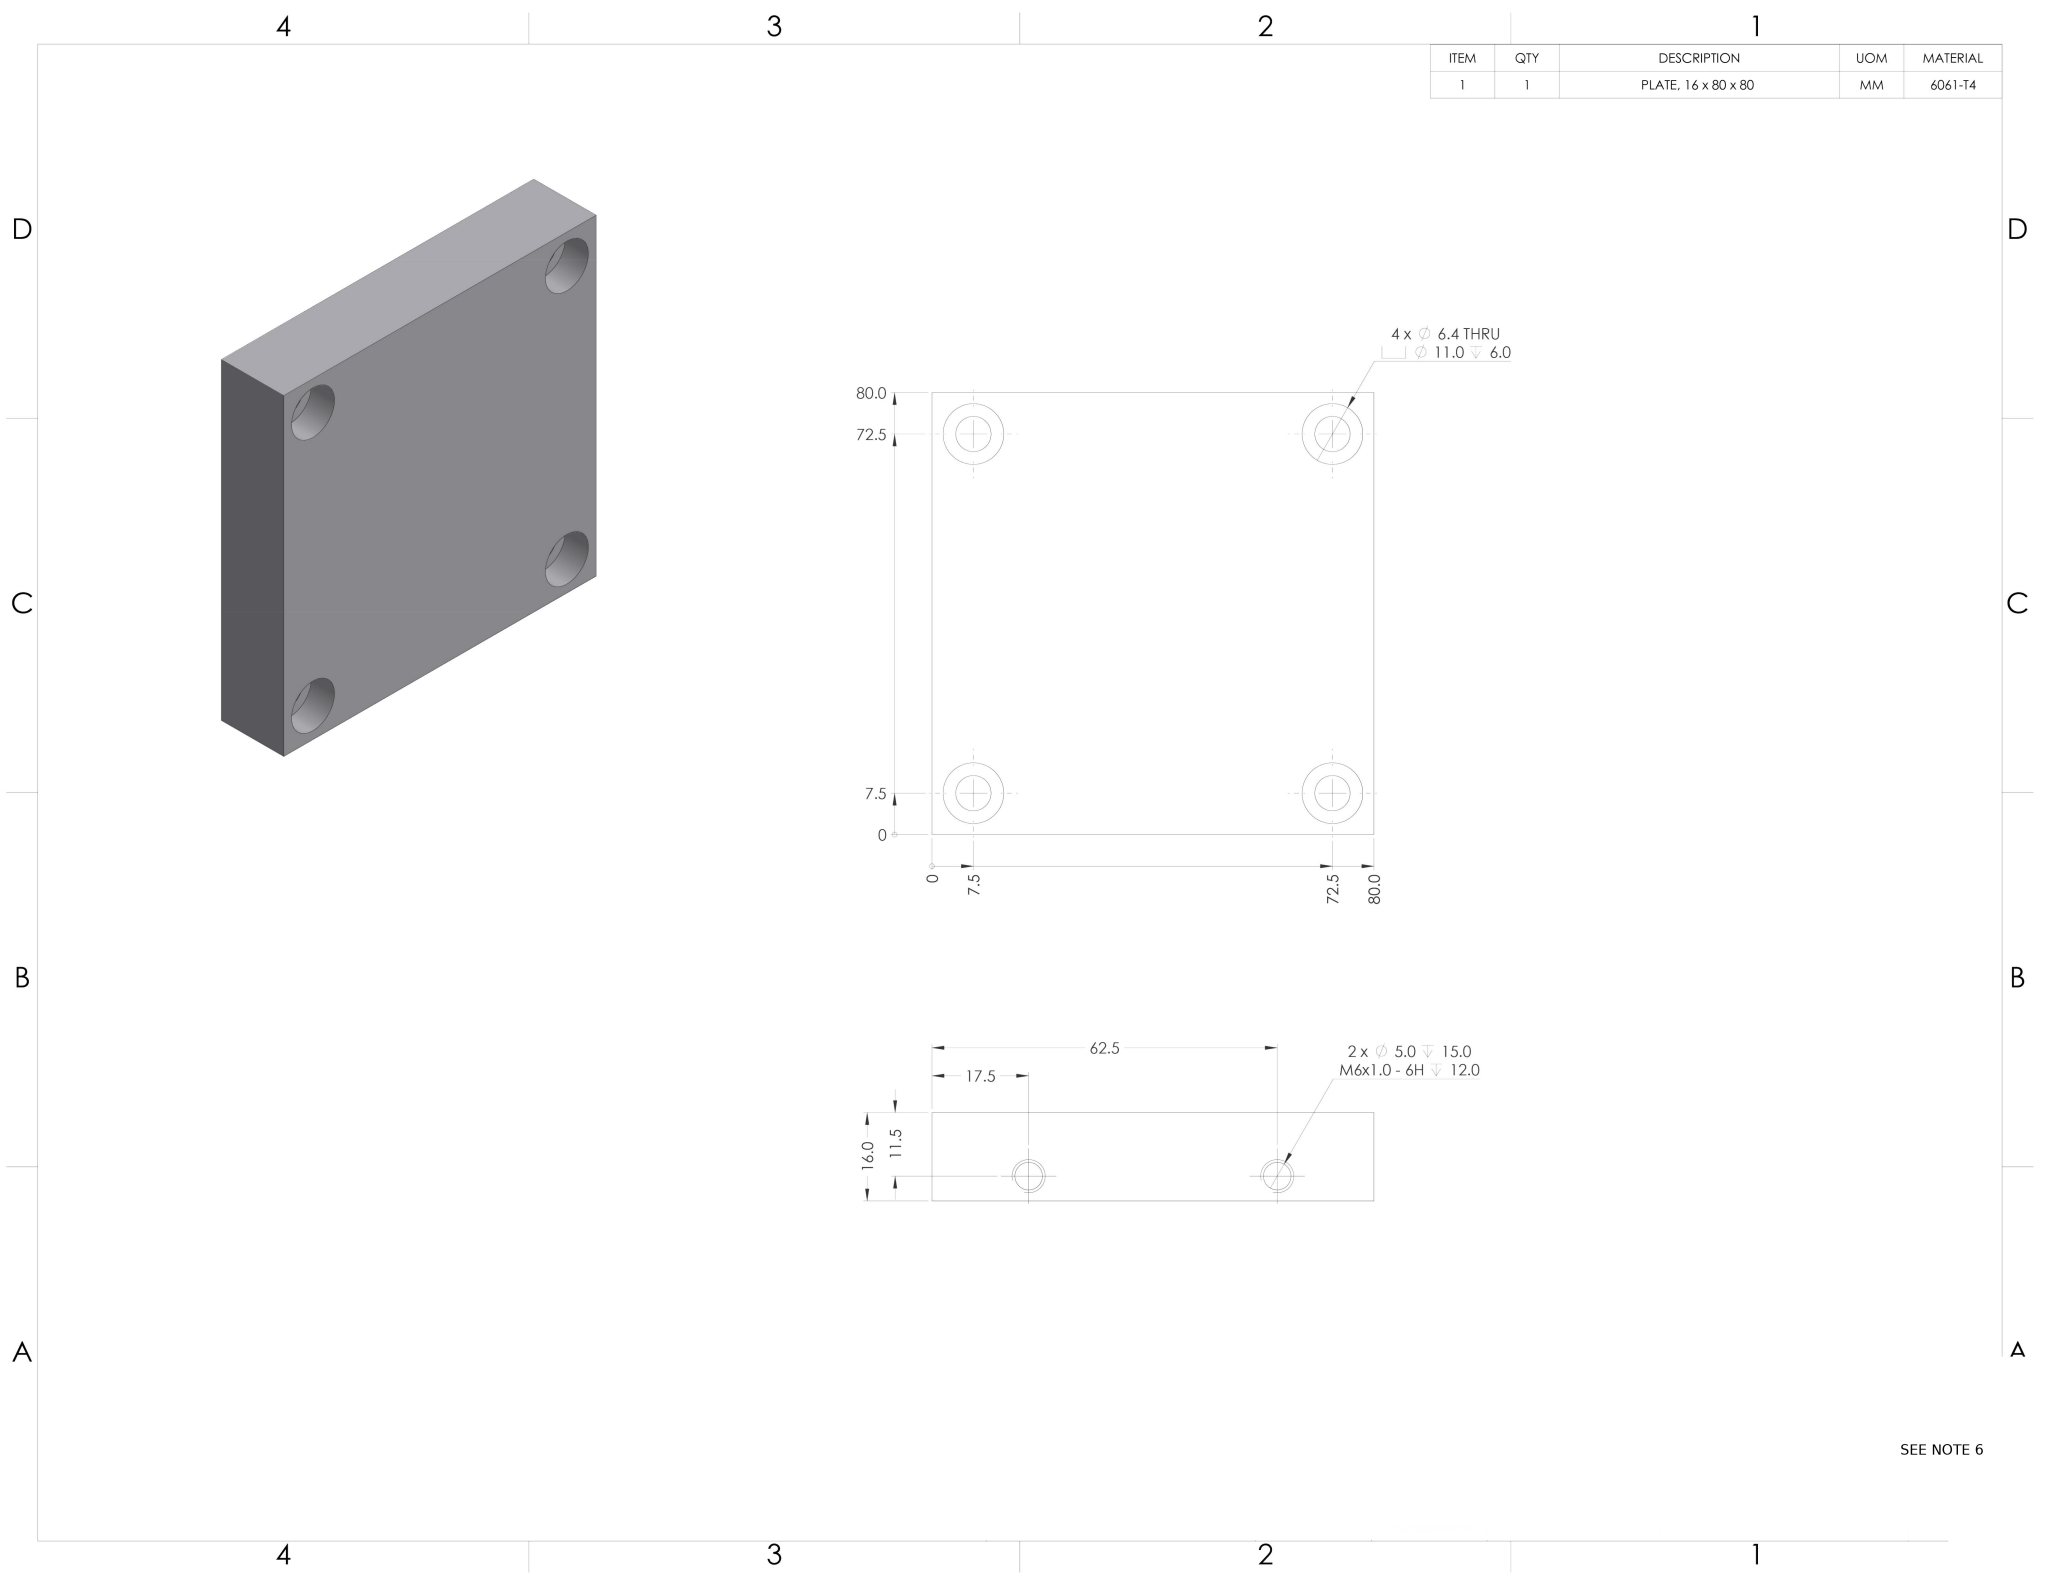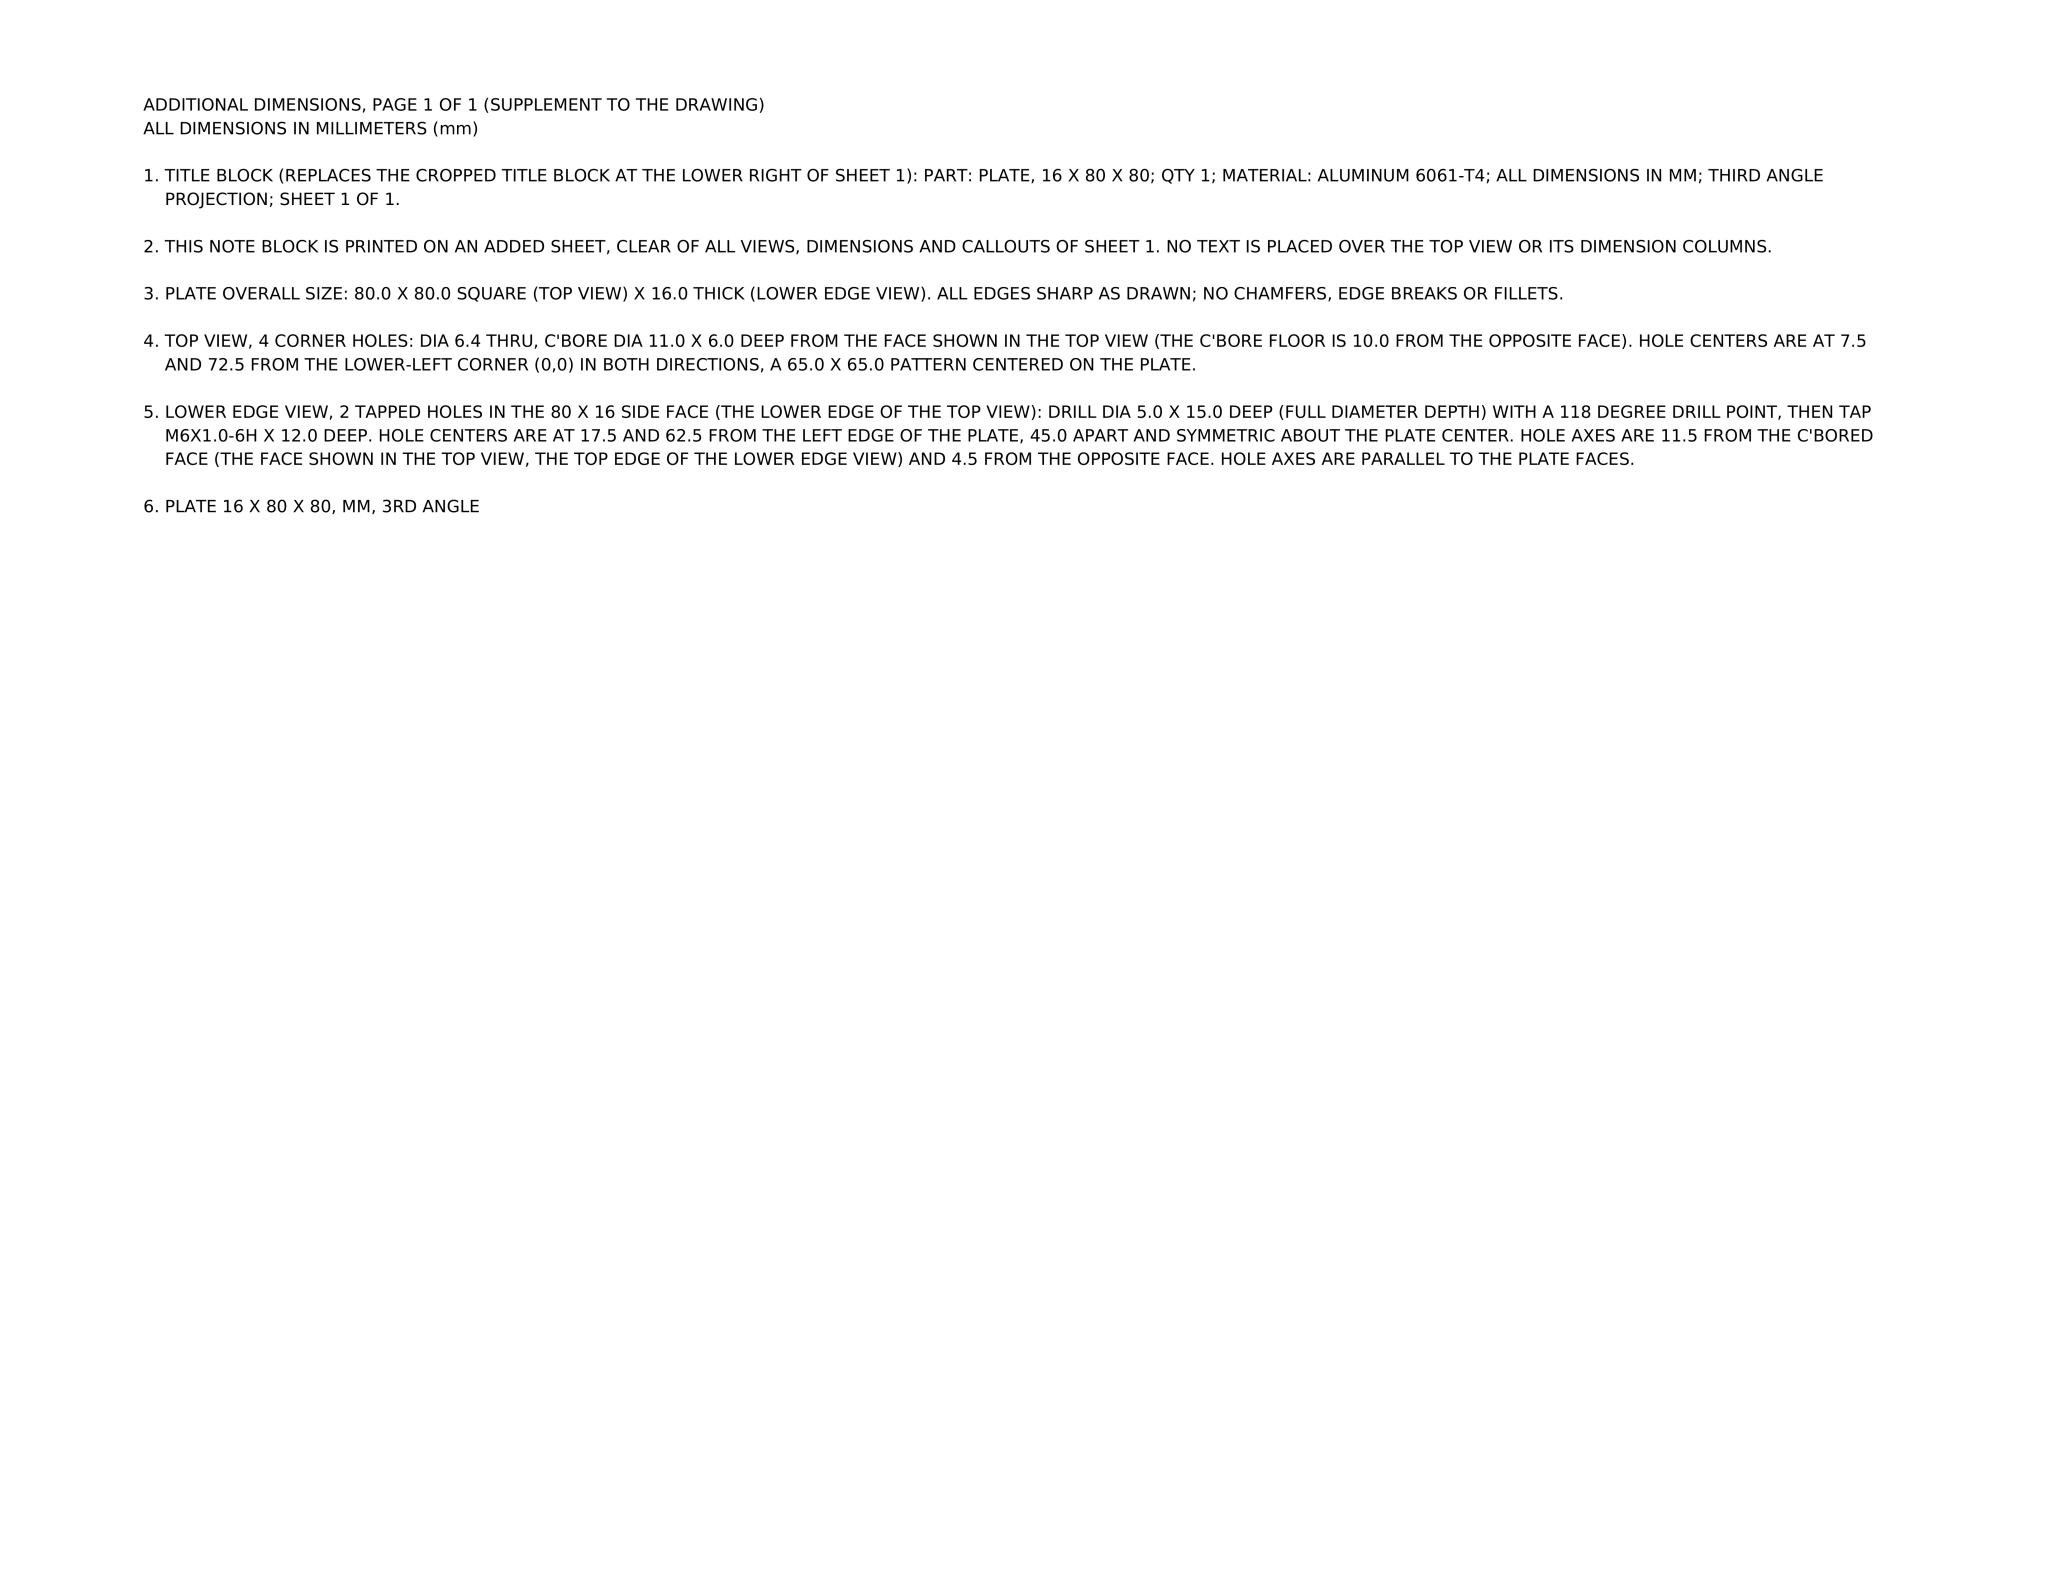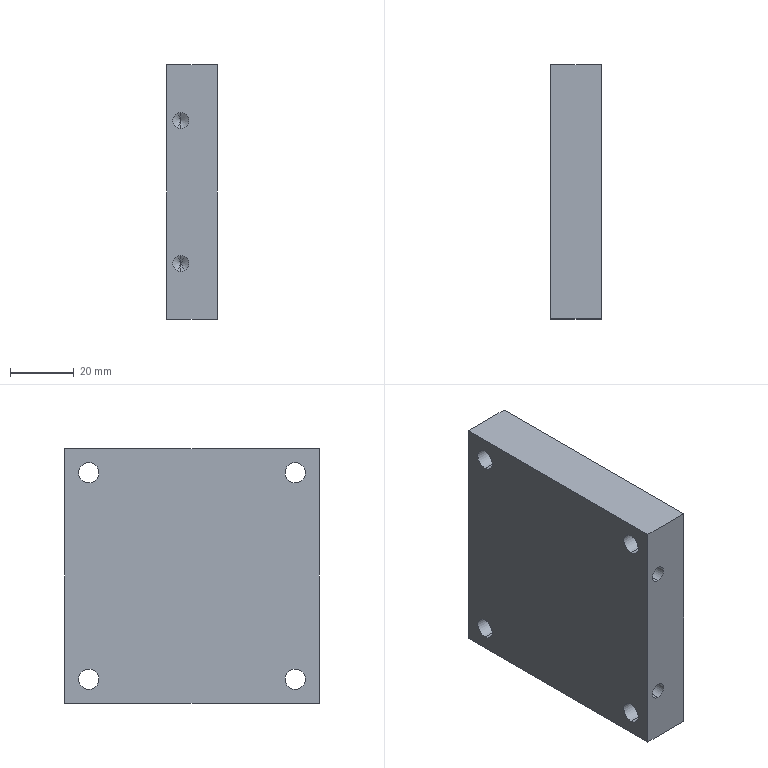Part | NX | mm | 1 solid | 34 faces | box 16 x 80 x 80 mm | volume 98224 mm3 | cylinder 20 | plane 10 | cone 4 | commonest cylinder face diameters 11 x8 6.4 x8 5 x4